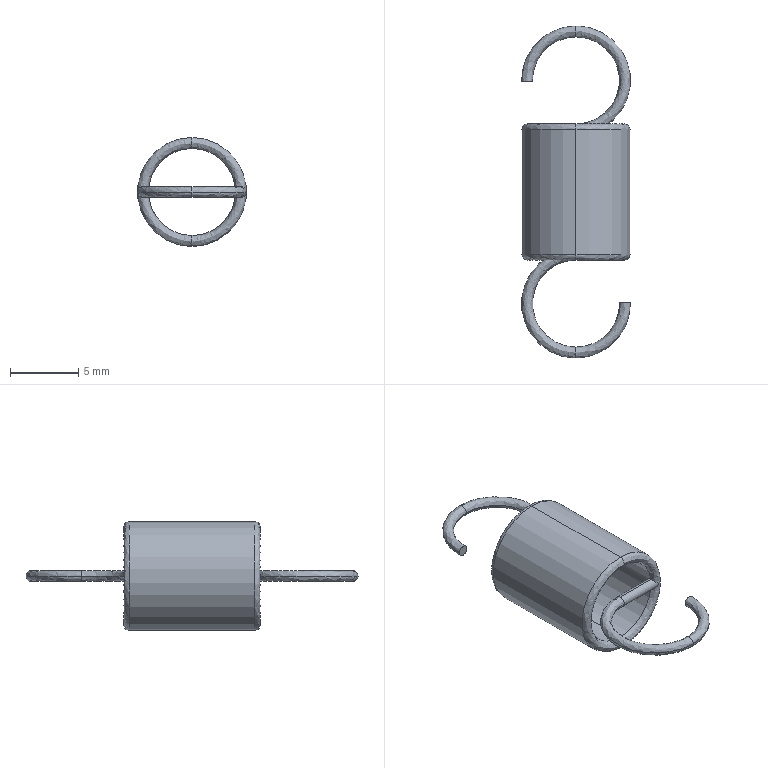Component | SolidWorks | LD101-02-WFSP8-0.8-10-2-6 | 1 solid | 22 faces | volume 198 mm3 | spline 12 | cylinder 8 | plane 2 | commonest cylinder face diameters 0.8 x4 8 x2 6.4 x2